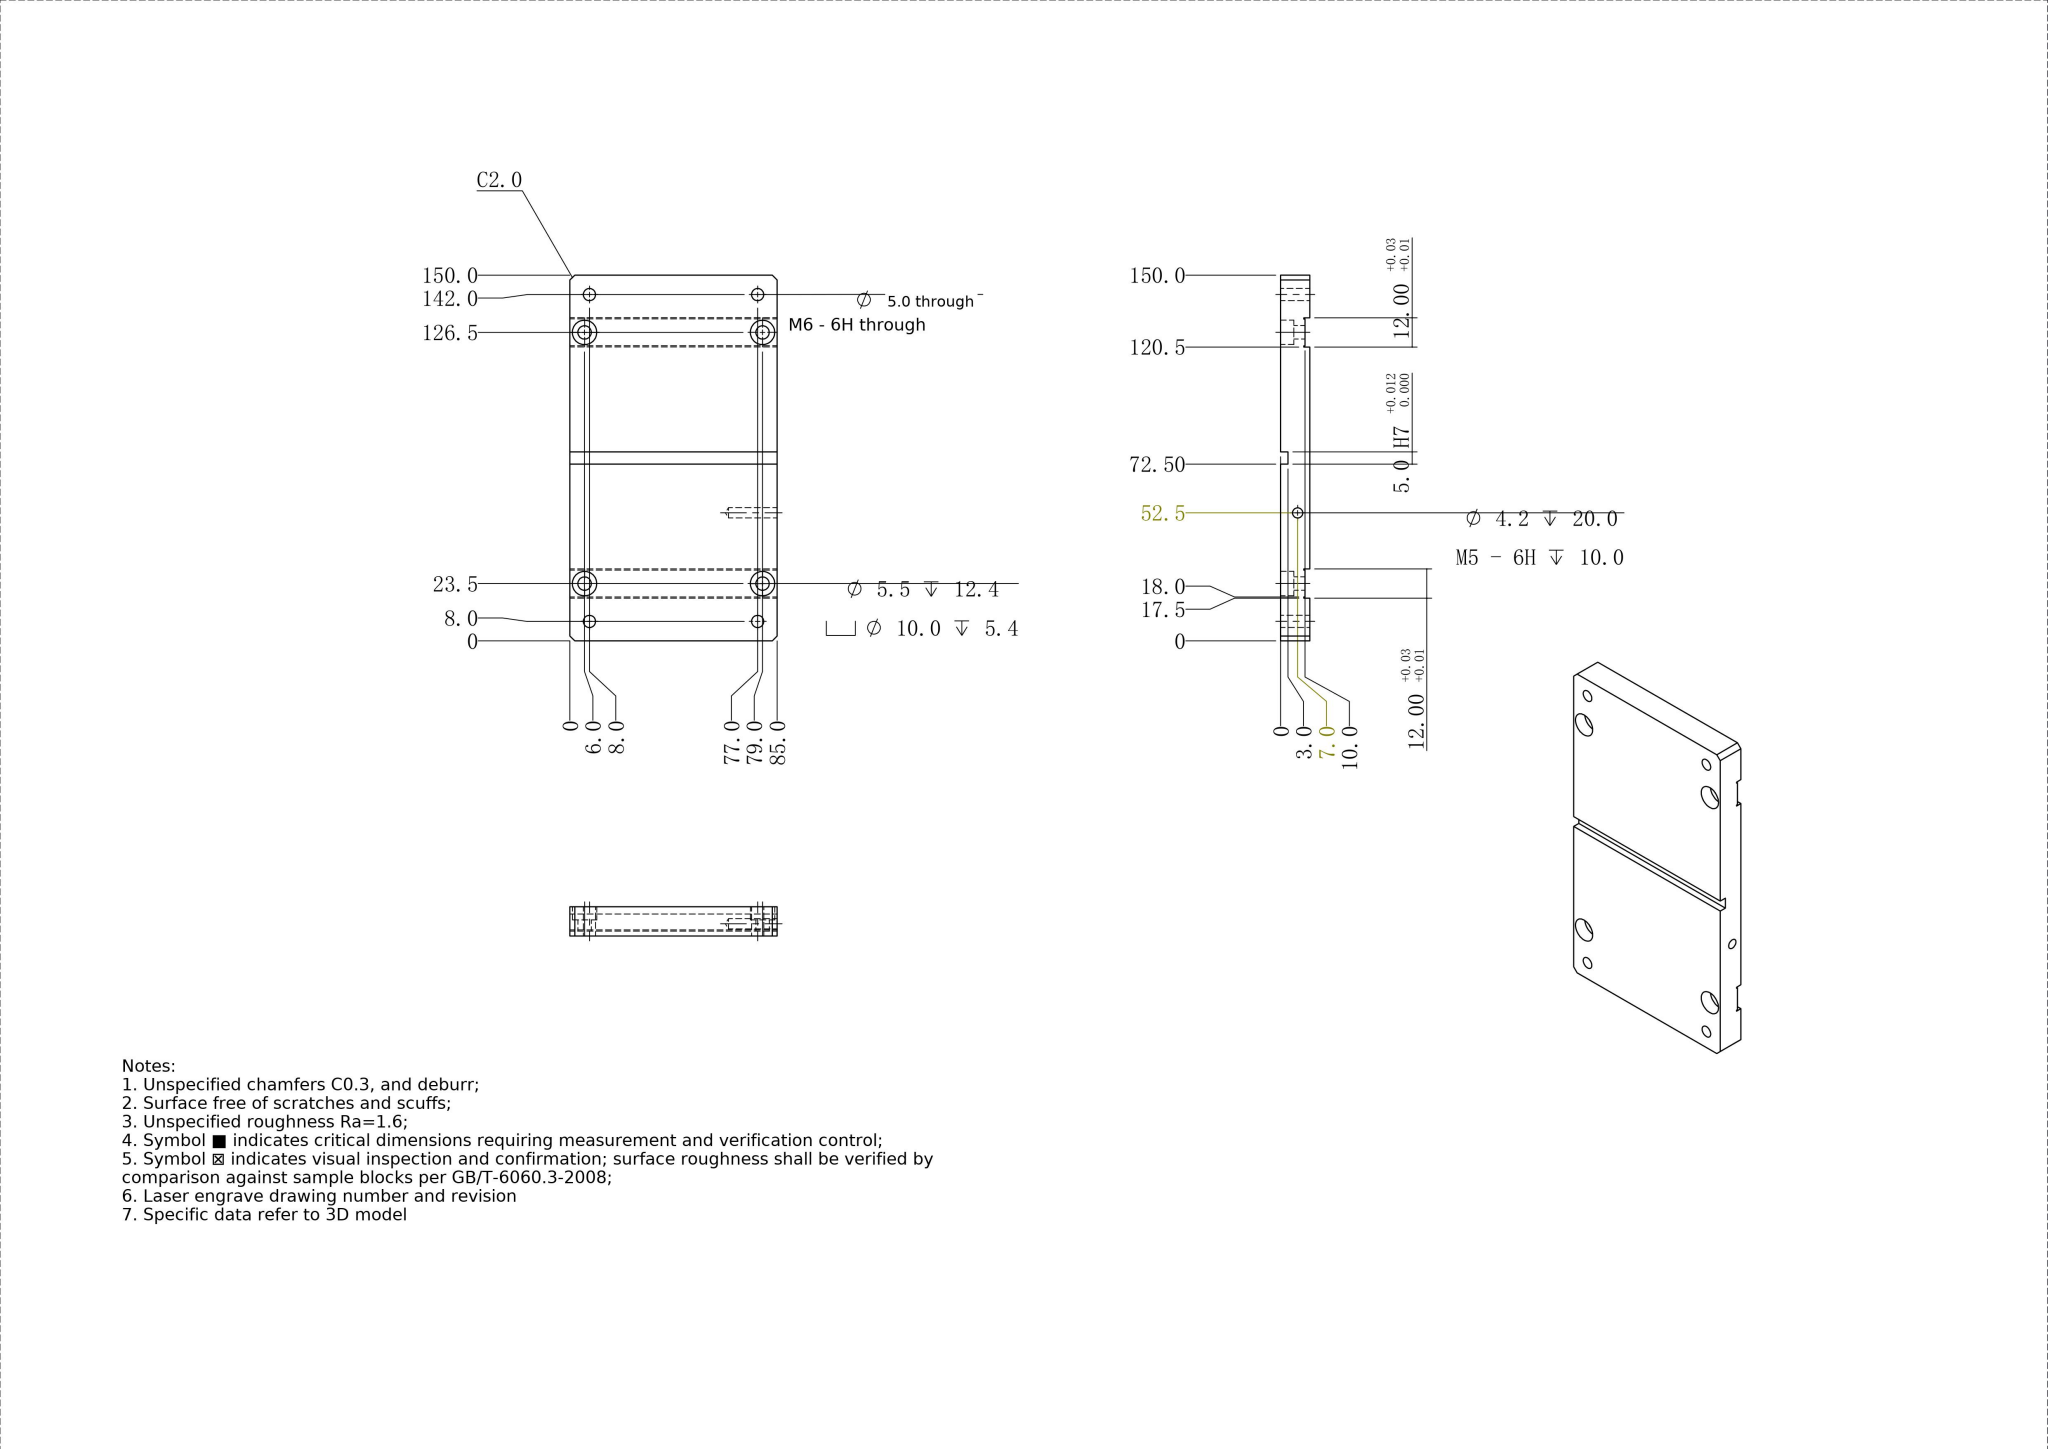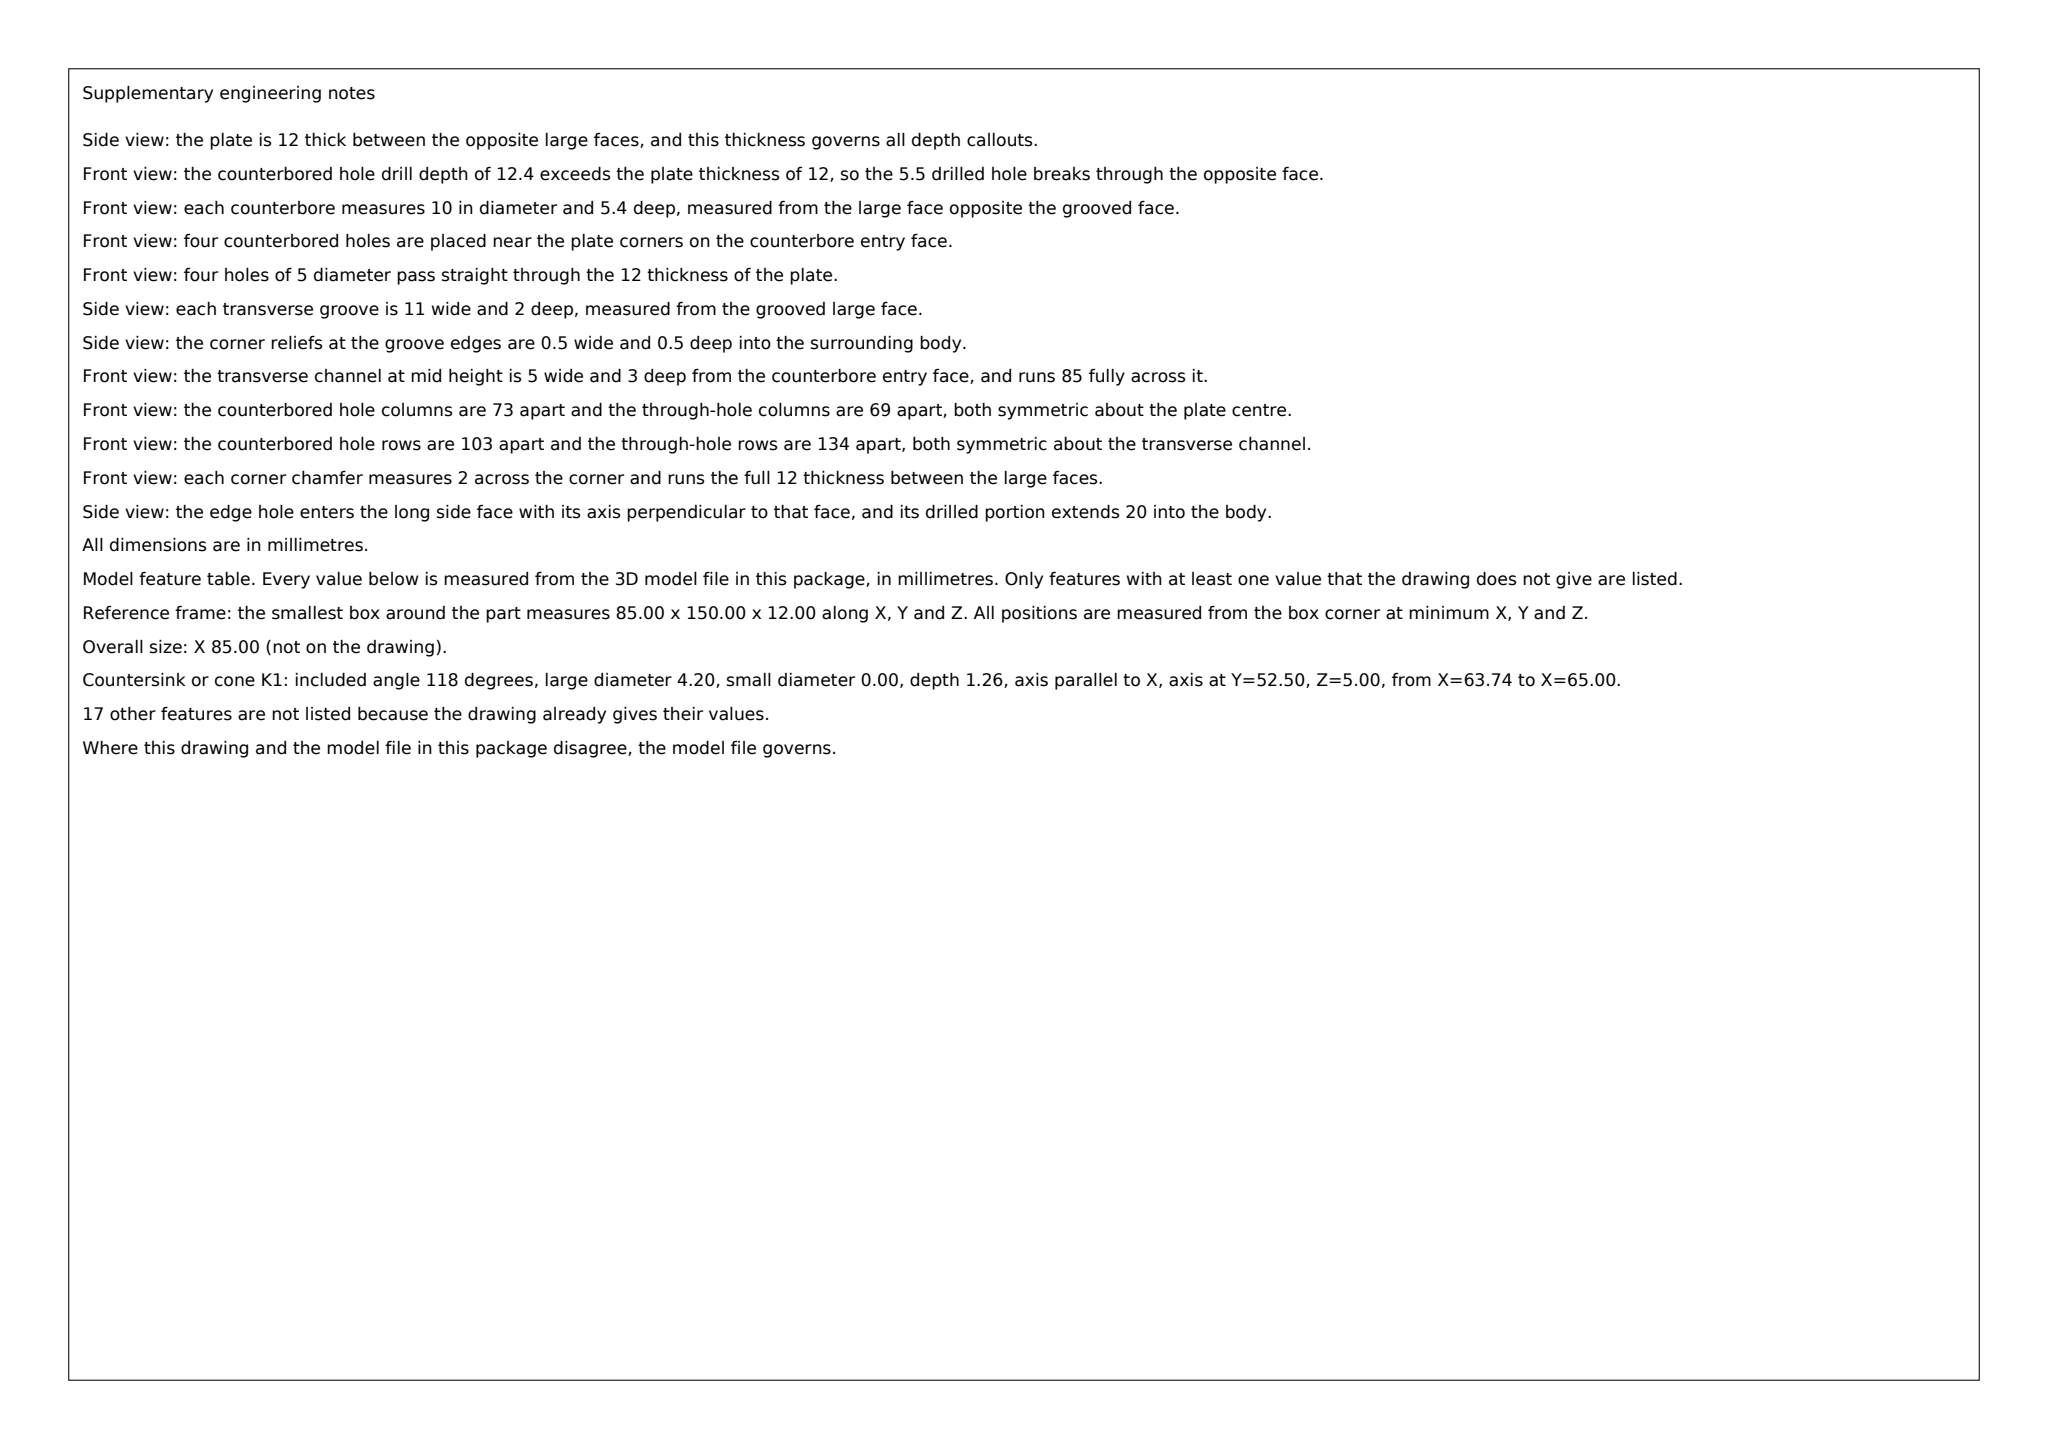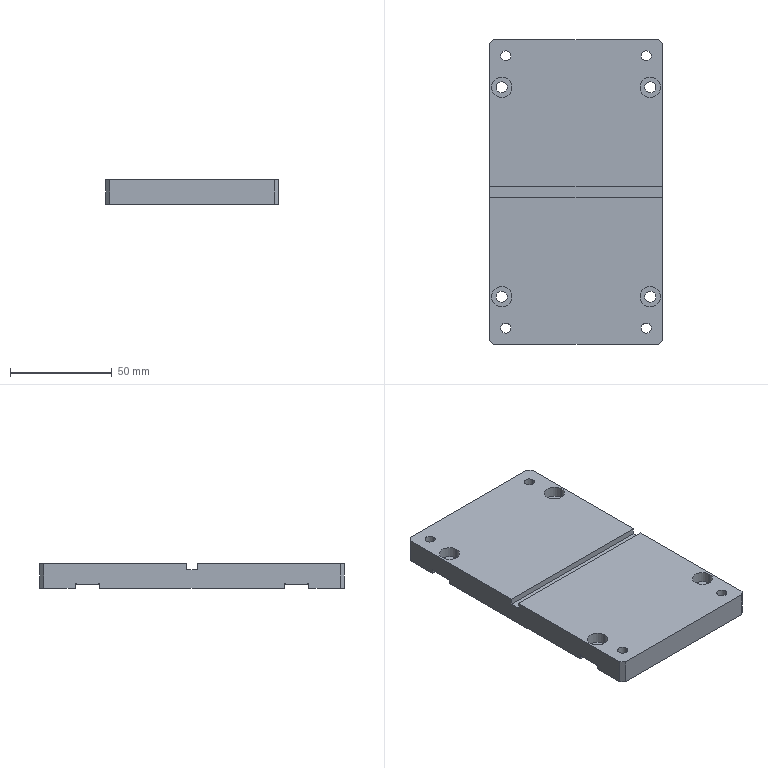Part | SolidWorks | mm | 1 solid | 62 faces | box 85 x 150 x 12 mm | volume 144105 mm3 | plane 34 | cylinder 26 | cone 2 | commonest cylinder face diameters 10 x8 5.5 x8 5 x8 4.2 x2
build123d program:
from build123d import *

# Parameters (mm, degrees)
SKETCH1_W                                       = 85
SKETCH1_H                                       = 150
BOSS_EXTRUDE1_DEPTH                             = 6
CHAMFER1_SIZE                                   = 2
SKETCH2_W                                       = 85
SKETCH2_H                                       = 12
CUT_EXTRUDE1_DEPTH                              = 2
M6_TAPPED_HOLE1_D                               = 5
SKETCH5_W                                       = 6
SKETCH5_H                                       = 5
CUT_EXTRUDE2_DEPTH                              = 207
M5_TAPPED_HOLE2_D                               = 4.2
M5_TAPPED_HOLE2_DEPTH                           = 20
M5_TAPPED_HOLE2_TIP                             = 1.262
M5_HEX_SOCKET_HEAD_CAP_SCREW_CBORE1_D           = 5.5
M5_HEX_SOCKET_HEAD_CAP_SCREW_CBORE1_DEPTH       = 12.4
M5_HEX_SOCKET_HEAD_CAP_SCREW_CBORE1_CBORE_D     = 10
M5_HEX_SOCKET_HEAD_CAP_SCREW_CBORE1_CBORE_DEPTH = 5.4
M5_HEX_SOCKET_HEAD_CAP_SCREW_CBORE1_TIP         = 1.652
SKETCH12_W                                      = 0.5
SKETCH12_H                                      = 0.5
CUT_EXTRUDE3_DEPTH                              = 206


with BuildPart() as part:
    # Sketch1 → Boss-Extrude1 (new, symmetric)
    with BuildSketch(Plane.XY):
        Rectangle(SKETCH1_W, SKETCH1_H)
    extrude(amount=BOSS_EXTRUDE1_DEPTH, both=True)

    # Chamfer1
    chamfer1_edges = [part.edges().sort_by_distance(p)[0] for p in [
        (42.5, -75, 0),
        (-42.5, -75, 0),
        (-42.5, 75, 0),
        (42.5, 75, 0),
    ]]
    chamfer(chamfer1_edges, length=CHAMFER1_SIZE)

    # Sketch2 → Cut-Extrude1 (cut)
    with BuildSketch(Plane(origin=(0, 0, -6), x_dir=(-1, 0, 0), z_dir=(0, 0, -1))):
        with Locations((0, 51.5)):
            Rectangle(SKETCH2_W, SKETCH2_H)
        with Locations((0, -51.5)):
            Rectangle(SKETCH2_W, SKETCH2_H)
    extrude(amount=-CUT_EXTRUDE1_DEPTH, mode=Mode.SUBTRACT)

    # M6 Tapped Hole1 (through all)
    with Locations(Plane(origin=(0, 0, -6), x_dir=(-1, 0, 0), z_dir=(0, 0, -1))):
        with Locations((-34.5, 67), (34.5, 67), (-34.5, -67), (34.5, -67)):
            Hole(M6_TAPPED_HOLE1_D / 2)

    # Sketch5 → Cut-Extrude2 (cut)
    with BuildSketch(Plane.ZY.offset(42.5)):
        with Locations((6, 0)):
            Rectangle(SKETCH5_W, SKETCH5_H)
    extrude(amount=-CUT_EXTRUDE2_DEPTH, mode=Mode.SUBTRACT)

    # M5 Tapped Hole2
    with Locations(Plane(origin=(42.5, 0, 0), x_dir=(0, 0, -1), z_dir=(1, 0, 0))):
        with Locations((1, -22.5)):
            Hole(M5_TAPPED_HOLE2_D / 2, depth=M5_TAPPED_HOLE2_DEPTH)
            with Locations((0, 0, -(M5_TAPPED_HOLE2_DEPTH + M5_TAPPED_HOLE2_TIP / 2))):  # 118° drill point
                Cone(0, M5_TAPPED_HOLE2_D / 2, M5_TAPPED_HOLE2_TIP, mode=Mode.SUBTRACT)

    # M5 Hex Socket Head Cap Screw CBORE1
    with Locations(Plane.XY.offset(6)):
        with Locations((36.5, 51.5), (-36.5, 51.5), (36.5, -51.5), (-36.5, -51.5)):
            CounterBoreHole(M5_HEX_SOCKET_HEAD_CAP_SCREW_CBORE1_D / 2, M5_HEX_SOCKET_HEAD_CAP_SCREW_CBORE1_CBORE_D / 2, M5_HEX_SOCKET_HEAD_CAP_SCREW_CBORE1_CBORE_DEPTH, depth=M5_HEX_SOCKET_HEAD_CAP_SCREW_CBORE1_DEPTH)
            with Locations((0, 0, -(M5_HEX_SOCKET_HEAD_CAP_SCREW_CBORE1_DEPTH + M5_HEX_SOCKET_HEAD_CAP_SCREW_CBORE1_TIP / 2))):  # 118° drill point
                Cone(0, M5_HEX_SOCKET_HEAD_CAP_SCREW_CBORE1_D / 2, M5_HEX_SOCKET_HEAD_CAP_SCREW_CBORE1_TIP, mode=Mode.SUBTRACT)

    # Sketch12 → Cut-Extrude3 (cut)
    with BuildSketch(Plane(origin=(42.5, 0, 0), x_dir=(0, 0, -1), z_dir=(1, 0, 0))):
        with Locations((3.75, 57.25)):
            Rectangle(SKETCH12_W, SKETCH12_H)
        with Locations((3.75, 45.75)):
            Rectangle(SKETCH12_W, SKETCH12_H)
        with Locations((3.75, -45.75)):
            Rectangle(SKETCH12_W, SKETCH12_H)
        with Locations((3.75, -57.25)):
            Rectangle(SKETCH12_W, SKETCH12_H)
    extrude(amount=-CUT_EXTRUDE3_DEPTH, mode=Mode.SUBTRACT)


solid = part.part